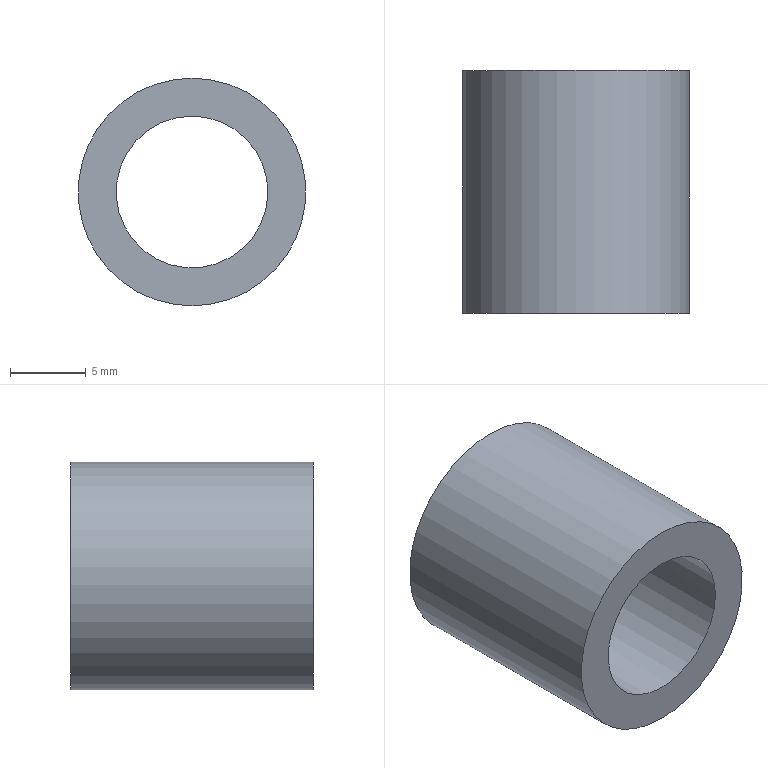Component | NX | JJZ-007 | 1 solid | 4 faces | box 15 x 16 x 15 mm | volume 1571 mm3 | plane 2 | cylinder 2 | commonest cylinder face diameters 15 x1 10 x1
STEP:
#1=CARTESIAN_POINT('',(0.,0.,0.));
#2=DIRECTION('',(0.,0.,1.));
#3=DIRECTION('',(1.,0.,0.));
#4=AXIS2_PLACEMENT_3D('',#1,#2,#3);
#5=CARTESIAN_POINT('',(32.529,4.,104.102));
#6=VERTEX_POINT('',#5);
#7=CARTESIAN_POINT('',(26.25,4.,100.));
#8=DIRECTION('',(0.,1.,0.));
#9=DIRECTION('',(0.8372,0.,0.5469));
#10=AXIS2_PLACEMENT_3D('',#7,#8,#9);
#11=CIRCLE('',#10,7.5);
#12=CARTESIAN_POINT('',(26.25,4.,100.));
#13=DIRECTION('',(0.,-1.,0.));
#14=DIRECTION('',(-0.8372,0.,-0.5469));
#15=AXIS2_PLACEMENT_3D('',#12,#13,#14);
#16=PLANE('',#15);
#17=CARTESIAN_POINT('',(-7.5,0.));
#18=CARTESIAN_POINT('',(-7.5,12.99));
#19=CARTESIAN_POINT('',(3.75,6.495));
#20=CARTESIAN_POINT('',(15.,0.));
#21=CARTESIAN_POINT('',(3.75,-6.495));
#22=CARTESIAN_POINT('',(-7.5,-12.99));
#23=CARTESIAN_POINT('',(-7.5,0.));
#24=(BOUNDED_CURVE()B_SPLINE_CURVE(2,(#17,#18,#19,#20,#21,#22,#23),.UNSPECIFIED.,.T.,.F.)B_SPLINE_CURVE_WITH_KNOTS((1,2,2,2,2,1),(-2.094,0.,2.094,4.189,6.283,8.378),.UNSPECIFIED.)CURVE()GEOMETRIC_REPRESENTATION_ITEM()RATIONAL_B_SPLINE_CURVE((1.,0.5,1.,0.5,1.,0.5,1.))REPRESENTATION_ITEM(''));
#25=(GEOMETRIC_REPRESENTATION_CONTEXT(2)PARAMETRIC_REPRESENTATION_CONTEXT()REPRESENTATION_CONTEXT('',''));
#26=DEFINITIONAL_REPRESENTATION('',(#24),#25);
#27=PCURVE('',#16,#26);
#28=CARTESIAN_POINT('',(26.25,4.,100.));
#29=DIRECTION('',(0.,1.,0.));
#30=DIRECTION('',(0.8372,0.,0.5469));
#31=AXIS2_PLACEMENT_3D('',#28,#29,#30);
#32=CYLINDRICAL_SURFACE('',#31,7.5);
#33=CARTESIAN_POINT('',(0.,0.));
#34=DIRECTION('',(1.,0.));
#35=VECTOR('',#34,1.);
#36=LINE('',#33,#35);
#37=(GEOMETRIC_REPRESENTATION_CONTEXT(2)PARAMETRIC_REPRESENTATION_CONTEXT()REPRESENTATION_CONTEXT('',''));
#38=DEFINITIONAL_REPRESENTATION('',(#36),#37);
#39=PCURVE('',#32,#38);
#40=SURFACE_CURVE('',#11,(#27,#39),.PCURVE_S1.);
#41=EDGE_CURVE('',#6,#6,#40,.T.);
#42=ORIENTED_EDGE('',*,*,#41,.F.);
#43=EDGE_LOOP('',(#42));
#44=FACE_BOUND('',#43,.T.);
#45=CARTESIAN_POINT('',(30.436,4.,102.735));
#46=VERTEX_POINT('',#45);
#47=CARTESIAN_POINT('',(26.25,4.,100.));
#48=DIRECTION('',(0.,1.,0.));
#49=DIRECTION('',(0.8372,0.,0.5469));
#50=AXIS2_PLACEMENT_3D('',#47,#48,#49);
#51=CIRCLE('',#50,5.);
#52=CARTESIAN_POINT('',(-5.,0.));
#53=CARTESIAN_POINT('',(-5.,8.66));
#54=CARTESIAN_POINT('',(2.5,4.33));
#55=CARTESIAN_POINT('',(10.,0.));
#56=CARTESIAN_POINT('',(2.5,-4.33));
#57=CARTESIAN_POINT('',(-5.,-8.66));
#58=CARTESIAN_POINT('',(-5.,0.));
#59=(BOUNDED_CURVE()B_SPLINE_CURVE(2,(#52,#53,#54,#55,#56,#57,#58),.UNSPECIFIED.,.T.,.F.)B_SPLINE_CURVE_WITH_KNOTS((1,2,2,2,2,1),(-2.094,0.,2.094,4.189,6.283,8.378),.UNSPECIFIED.)CURVE()GEOMETRIC_REPRESENTATION_ITEM()RATIONAL_B_SPLINE_CURVE((1.,0.5,1.,0.5,1.,0.5,1.))REPRESENTATION_ITEM(''));
#60=(GEOMETRIC_REPRESENTATION_CONTEXT(2)PARAMETRIC_REPRESENTATION_CONTEXT()REPRESENTATION_CONTEXT('',''));
#61=DEFINITIONAL_REPRESENTATION('',(#59),#60);
#62=PCURVE('',#16,#61);
#63=CARTESIAN_POINT('',(26.25,4.,100.));
#64=DIRECTION('',(0.,1.,0.));
#65=DIRECTION('',(0.8372,0.,0.5469));
#66=AXIS2_PLACEMENT_3D('',#63,#64,#65);
#67=CYLINDRICAL_SURFACE('',#66,5.);
#68=CARTESIAN_POINT('',(0.,0.));
#69=DIRECTION('',(1.,0.));
#70=VECTOR('',#69,1.);
#71=LINE('',#68,#70);
#72=(GEOMETRIC_REPRESENTATION_CONTEXT(2)PARAMETRIC_REPRESENTATION_CONTEXT()REPRESENTATION_CONTEXT('',''));
#73=DEFINITIONAL_REPRESENTATION('',(#71),#72);
#74=PCURVE('',#67,#73);
#75=SURFACE_CURVE('',#51,(#62,#74),.PCURVE_S1.);
#76=EDGE_CURVE('',#46,#46,#75,.T.);
#77=ORIENTED_EDGE('',*,*,#76,.T.);
#78=EDGE_LOOP('',(#77));
#79=FACE_BOUND('',#78,.T.);
#80=ADVANCED_FACE('',(#44,#79),#16,.T.);
#81=CARTESIAN_POINT('',(32.529,20.,104.102));
#82=VERTEX_POINT('',#81);
#83=CARTESIAN_POINT('',(26.25,20.,100.));
#84=DIRECTION('',(0.,1.,0.));
#85=DIRECTION('',(0.8372,0.,0.5469));
#86=AXIS2_PLACEMENT_3D('',#83,#84,#85);
#87=CIRCLE('',#86,7.5);
#88=CARTESIAN_POINT('',(26.25,20.,100.));
#89=DIRECTION('',(0.,-1.,0.));
#90=DIRECTION('',(-0.8372,0.,-0.5469));
#91=AXIS2_PLACEMENT_3D('',#88,#89,#90);
#92=PLANE('',#91);
#93=CARTESIAN_POINT('',(-7.5,0.));
#94=CARTESIAN_POINT('',(-7.5,12.99));
#95=CARTESIAN_POINT('',(3.75,6.495));
#96=CARTESIAN_POINT('',(15.,0.));
#97=CARTESIAN_POINT('',(3.75,-6.495));
#98=CARTESIAN_POINT('',(-7.5,-12.99));
#99=CARTESIAN_POINT('',(-7.5,0.));
#100=(BOUNDED_CURVE()B_SPLINE_CURVE(2,(#93,#94,#95,#96,#97,#98,#99),.UNSPECIFIED.,.T.,.F.)B_SPLINE_CURVE_WITH_KNOTS((1,2,2,2,2,1),(-2.094,0.,2.094,4.189,6.283,8.378),.UNSPECIFIED.)CURVE()GEOMETRIC_REPRESENTATION_ITEM()RATIONAL_B_SPLINE_CURVE((1.,0.5,1.,0.5,1.,0.5,1.))REPRESENTATION_ITEM(''));
#101=(GEOMETRIC_REPRESENTATION_CONTEXT(2)PARAMETRIC_REPRESENTATION_CONTEXT()REPRESENTATION_CONTEXT('',''));
#102=DEFINITIONAL_REPRESENTATION('',(#100),#101);
#103=PCURVE('',#92,#102);
#104=CARTESIAN_POINT('',(0.,16.));
#105=DIRECTION('',(1.,0.));
#106=VECTOR('',#105,1.);
#107=LINE('',#104,#106);
#108=(GEOMETRIC_REPRESENTATION_CONTEXT(2)PARAMETRIC_REPRESENTATION_CONTEXT()REPRESENTATION_CONTEXT('',''));
#109=DEFINITIONAL_REPRESENTATION('',(#107),#108);
#110=PCURVE('',#32,#109);
#111=SURFACE_CURVE('',#87,(#103,#110),.PCURVE_S1.);
#112=EDGE_CURVE('',#82,#82,#111,.T.);
#113=ORIENTED_EDGE('',*,*,#112,.T.);
#114=EDGE_LOOP('',(#113));
#115=FACE_BOUND('',#114,.T.);
#116=CARTESIAN_POINT('',(30.436,20.,102.735));
#117=VERTEX_POINT('',#116);
#118=CARTESIAN_POINT('',(26.25,20.,100.));
#119=DIRECTION('',(0.,1.,0.));
#120=DIRECTION('',(0.8372,0.,0.5469));
#121=AXIS2_PLACEMENT_3D('',#118,#119,#120);
#122=CIRCLE('',#121,5.);
#123=CARTESIAN_POINT('',(-5.,0.));
#124=CARTESIAN_POINT('',(-5.,8.66));
#125=CARTESIAN_POINT('',(2.5,4.33));
#126=CARTESIAN_POINT('',(10.,0.));
#127=CARTESIAN_POINT('',(2.5,-4.33));
#128=CARTESIAN_POINT('',(-5.,-8.66));
#129=CARTESIAN_POINT('',(-5.,0.));
#130=(BOUNDED_CURVE()B_SPLINE_CURVE(2,(#123,#124,#125,#126,#127,#128,#129),.UNSPECIFIED.,.T.,.F.)B_SPLINE_CURVE_WITH_KNOTS((1,2,2,2,2,1),(-2.094,0.,2.094,4.189,6.283,8.378),.UNSPECIFIED.)CURVE()GEOMETRIC_REPRESENTATION_ITEM()RATIONAL_B_SPLINE_CURVE((1.,0.5,1.,0.5,1.,0.5,1.))REPRESENTATION_ITEM(''));
#131=(GEOMETRIC_REPRESENTATION_CONTEXT(2)PARAMETRIC_REPRESENTATION_CONTEXT()REPRESENTATION_CONTEXT('',''));
#132=DEFINITIONAL_REPRESENTATION('',(#130),#131);
#133=PCURVE('',#92,#132);
#134=CARTESIAN_POINT('',(0.,16.));
#135=DIRECTION('',(1.,0.));
#136=VECTOR('',#135,1.);
#137=LINE('',#134,#136);
#138=(GEOMETRIC_REPRESENTATION_CONTEXT(2)PARAMETRIC_REPRESENTATION_CONTEXT()REPRESENTATION_CONTEXT('',''));
#139=DEFINITIONAL_REPRESENTATION('',(#137),#138);
#140=PCURVE('',#67,#139);
#141=SURFACE_CURVE('',#122,(#133,#140),.PCURVE_S1.);
#142=EDGE_CURVE('',#117,#117,#141,.T.);
#143=ORIENTED_EDGE('',*,*,#142,.F.);
#144=EDGE_LOOP('',(#143));
#145=FACE_BOUND('',#144,.T.);
#146=ADVANCED_FACE('',(#115,#145),#92,.F.);
#147=ORIENTED_EDGE('',*,*,#41,.T.);
#148=CARTESIAN_POINT('',(32.529,4.,104.102));
#149=CARTESIAN_POINT('',(32.529,20.,104.102));
#150=B_SPLINE_CURVE_WITH_KNOTS('',1,(#148,#149),.UNSPECIFIED.,.F.,.F.,(2,2),(0.,16.),.PIECEWISE_BEZIER_KNOTS.);
#151=CARTESIAN_POINT('',(6.283,0.));
#152=DIRECTION('',(0.,1.));
#153=VECTOR('',#152,1.);
#154=LINE('',#151,#153);
#155=(GEOMETRIC_REPRESENTATION_CONTEXT(2)PARAMETRIC_REPRESENTATION_CONTEXT()REPRESENTATION_CONTEXT('',''));
#156=DEFINITIONAL_REPRESENTATION('',(#154),#155);
#157=PCURVE('',#32,#156);
#158=CARTESIAN_POINT('',(0.,0.));
#159=DIRECTION('',(0.,1.));
#160=VECTOR('',#159,1.);
#161=LINE('',#158,#160);
#162=(GEOMETRIC_REPRESENTATION_CONTEXT(2)PARAMETRIC_REPRESENTATION_CONTEXT()REPRESENTATION_CONTEXT('',''));
#163=DEFINITIONAL_REPRESENTATION('',(#161),#162);
#164=PCURVE('',#32,#163);
#165=SEAM_CURVE('',#150,(#157,#164),.PCURVE_S1.);
#166=EDGE_CURVE('',#6,#82,#165,.T.);
#167=ORIENTED_EDGE('',*,*,#166,.T.);
#168=ORIENTED_EDGE('',*,*,#112,.F.);
#169=ORIENTED_EDGE('',*,*,#166,.F.);
#170=EDGE_LOOP('',(#147,#167,#168,#169));
#171=FACE_BOUND('',#170,.T.);
#172=ADVANCED_FACE('',(#171),#32,.T.);
#173=ORIENTED_EDGE('',*,*,#76,.T.);
#174=CARTESIAN_POINT('',(30.436,4.,102.735));
#175=CARTESIAN_POINT('',(30.436,20.,102.735));
#176=B_SPLINE_CURVE_WITH_KNOTS('',1,(#174,#175),.UNSPECIFIED.,.F.,.F.,(2,2),(0.,16.),.PIECEWISE_BEZIER_KNOTS.);
#177=CARTESIAN_POINT('',(6.283,0.));
#178=DIRECTION('',(0.,1.));
#179=VECTOR('',#178,1.);
#180=LINE('',#177,#179);
#181=(GEOMETRIC_REPRESENTATION_CONTEXT(2)PARAMETRIC_REPRESENTATION_CONTEXT()REPRESENTATION_CONTEXT('',''));
#182=DEFINITIONAL_REPRESENTATION('',(#180),#181);
#183=PCURVE('',#67,#182);
#184=CARTESIAN_POINT('',(0.,0.));
#185=DIRECTION('',(0.,1.));
#186=VECTOR('',#185,1.);
#187=LINE('',#184,#186);
#188=(GEOMETRIC_REPRESENTATION_CONTEXT(2)PARAMETRIC_REPRESENTATION_CONTEXT()REPRESENTATION_CONTEXT('',''));
#189=DEFINITIONAL_REPRESENTATION('',(#187),#188);
#190=PCURVE('',#67,#189);
#191=SEAM_CURVE('',#176,(#183,#190),.PCURVE_S1.);
#192=EDGE_CURVE('',#46,#117,#191,.T.);
#193=ORIENTED_EDGE('',*,*,#192,.T.);
#194=ORIENTED_EDGE('',*,*,#142,.F.);
#195=ORIENTED_EDGE('',*,*,#192,.F.);
#196=EDGE_LOOP('',(#173,#193,#194,#195));
#197=FACE_BOUND('',#196,.F.);
#198=ADVANCED_FACE('',(#197),#67,.F.);
#199=CLOSED_SHELL('',(#80,#146,#172,#198));
#200=MANIFOLD_SOLID_BREP('',#199);
#201=(LENGTH_UNIT()NAMED_UNIT(*)SI_UNIT(.MILLI.,.METRE.));
#202=UNCERTAINTY_MEASURE_WITH_UNIT(LENGTH_MEASURE(0.00001),#201,'','');
#203=(NAMED_UNIT(*)PLANE_ANGLE_UNIT()SI_UNIT($,.RADIAN.));
#204=(NAMED_UNIT(*)SI_UNIT($,.STERADIAN.)SOLID_ANGLE_UNIT());
#205=(GEOMETRIC_REPRESENTATION_CONTEXT(3)GLOBAL_UNCERTAINTY_ASSIGNED_CONTEXT((#202))GLOBAL_UNIT_ASSIGNED_CONTEXT((#201,#203,#204))REPRESENTATION_CONTEXT('',''));
#206=ADVANCED_BREP_SHAPE_REPRESENTATION('',(#4,#200),#205);